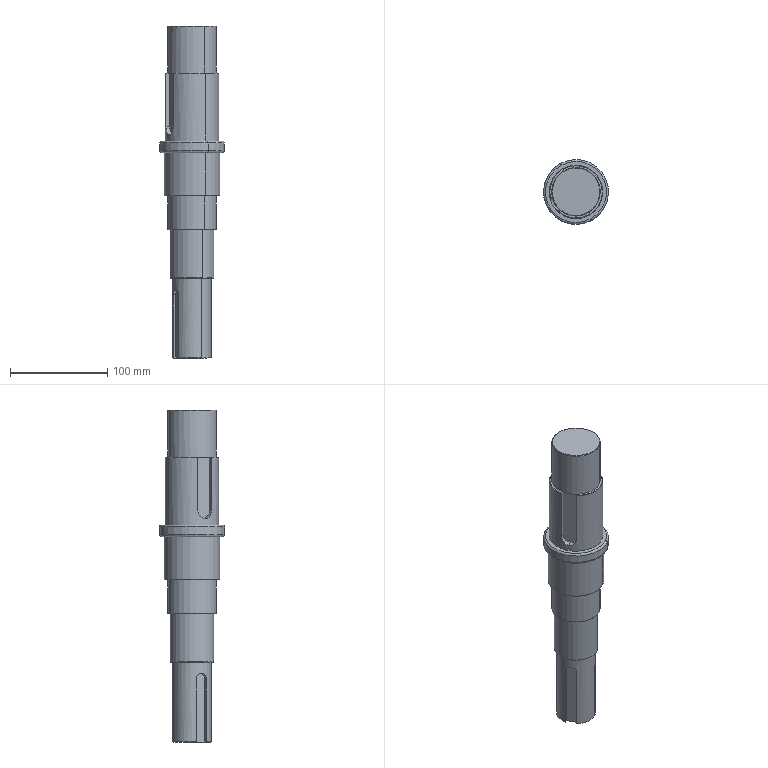Component | SolidWorks | OutputAxis0717-1 | 1 solid | 55 faces | volume 656767 mm3 | cylinder 20 | cone 16 | plane 15 | torus 4 | commonest cylinder face diameters 50 x4 10.2 x2 55 x2 67 x2 57 x2 45 x2 40 x2 12 x2